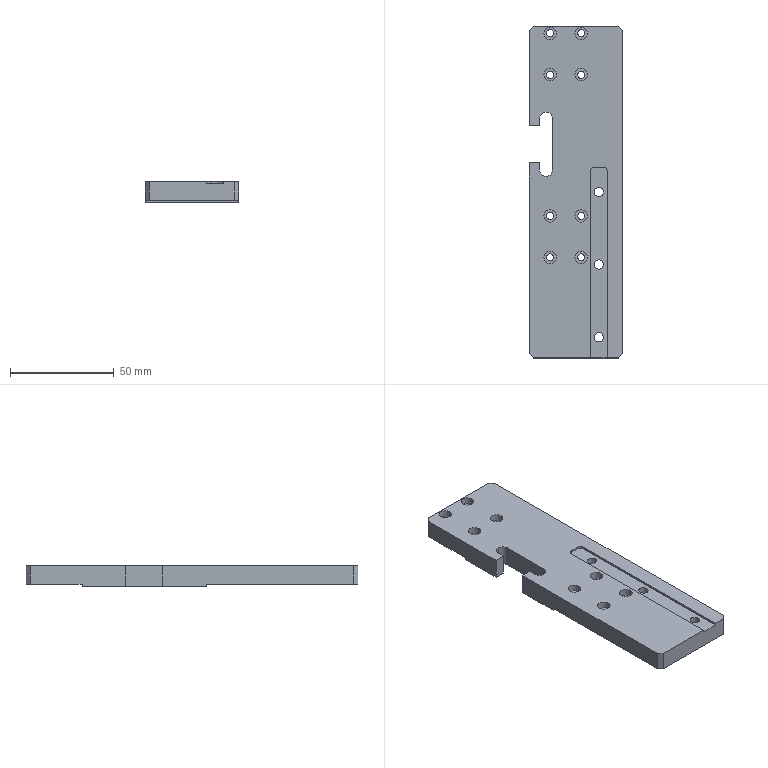Component | SolidWorks | 200-03-1 | 1 solid | 85 faces | box 45 x 160 x 10 mm | volume 61883 mm3 | cylinder 50 | plane 35 | commonest cylinder face diameters 6 x16 3.4 x16 8 x6 4.5 x6 6.2 x4 4 x2 | material 45